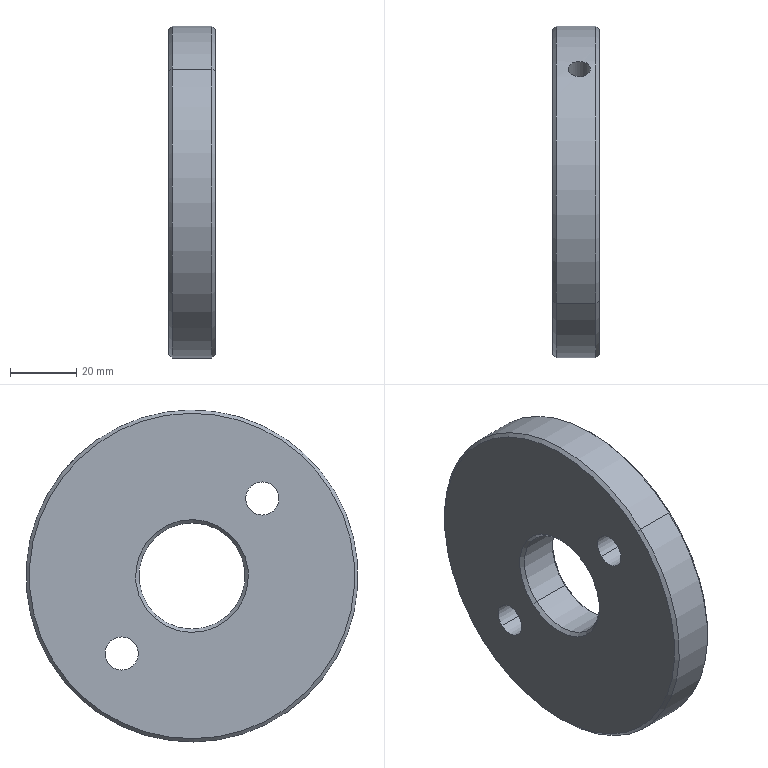Component | SolidWorks | 2-10-10WorkpieceAxisAssembly-1_Flange1-1 | 1 solid | 20 faces | box 14 x 100 x 100 mm | volume 94846 mm3 | cylinder 10 | cone 8 | plane 2 | commonest cylinder face diameters 10 x4 6.8 x2 32 x2 100 x2
STEP:
#1=COLOUR_RGB('',0.7922,0.8196,0.9333);
#2=FILL_AREA_STYLE_COLOUR('',#1);
#3=FILL_AREA_STYLE('',(#2));
#4=SURFACE_STYLE_FILL_AREA(#3);
#5=SURFACE_SIDE_STYLE('',(#4));
#6=SURFACE_STYLE_USAGE(.BOTH.,#5);
#7=PRESENTATION_STYLE_ASSIGNMENT((#6));
#8=CARTESIAN_POINT('',(-6.662,0.302,0.4232));
#9=VERTEX_POINT('',#8);
#10=CARTESIAN_POINT('',(-6.394,0.302,0.4232));
#11=VERTEX_POINT('',#10);
#12=CARTESIAN_POINT('',(-6.662,0.302,0.4232));
#13=CARTESIAN_POINT('',(-6.662,0.3079,0.4166));
#14=CARTESIAN_POINT('',(-6.661,0.3136,0.4101));
#15=CARTESIAN_POINT('',(-6.657,0.3246,0.3969));
#16=CARTESIAN_POINT('',(-6.655,0.33,0.3902));
#17=CARTESIAN_POINT('',(-6.648,0.3399,0.3773));
#18=CARTESIAN_POINT('',(-6.644,0.3444,0.3711));
#19=CARTESIAN_POINT('',(-6.634,0.3529,0.3592));
#20=CARTESIAN_POINT('',(-6.629,0.3568,0.3535));
#21=CARTESIAN_POINT('',(-6.616,0.3637,0.3431));
#22=CARTESIAN_POINT('',(-6.61,0.3667,0.3384));
#23=CARTESIAN_POINT('',(-6.595,0.372,0.3299));
#24=CARTESIAN_POINT('',(-6.587,0.3742,0.3263));
#25=CARTESIAN_POINT('',(-6.571,0.3777,0.3205));
#26=CARTESIAN_POINT('',(-6.563,0.379,0.3182));
#27=CARTESIAN_POINT('',(-6.545,0.3808,0.3152));
#28=CARTESIAN_POINT('',(-6.537,0.3812,0.3144));
#29=CARTESIAN_POINT('',(-6.519,0.3812,0.3144));
#30=CARTESIAN_POINT('',(-6.51,0.3808,0.3152));
#31=CARTESIAN_POINT('',(-6.493,0.379,0.3182));
#32=CARTESIAN_POINT('',(-6.485,0.3777,0.3205));
#33=CARTESIAN_POINT('',(-6.469,0.3742,0.3263));
#34=CARTESIAN_POINT('',(-6.461,0.372,0.33));
#35=CARTESIAN_POINT('',(-6.446,0.3668,0.3383));
#36=CARTESIAN_POINT('',(-6.439,0.3637,0.3431));
#37=CARTESIAN_POINT('',(-6.427,0.3568,0.3536));
#38=CARTESIAN_POINT('',(-6.422,0.3529,0.3592));
#39=CARTESIAN_POINT('',(-6.412,0.3445,0.371));
#40=CARTESIAN_POINT('',(-6.408,0.3398,0.3774));
#41=CARTESIAN_POINT('',(-6.401,0.3299,0.3903));
#42=CARTESIAN_POINT('',(-6.398,0.3247,0.3968));
#43=CARTESIAN_POINT('',(-6.395,0.3137,0.41));
#44=CARTESIAN_POINT('',(-6.394,0.3078,0.4167));
#45=CARTESIAN_POINT('',(-6.394,0.302,0.4232));
#46=B_SPLINE_CURVE_WITH_KNOTS('',3,(#12,#13,#14,#15,#16,#17,#18,#19,#20,#21,#22,#23,#24,#25,#26,#27,#28,#29,#30,#31,#32,#33,#34,#35,#36,#37,#38,#39,#40,#41,#42,#43,#44,#45),.UNSPECIFIED.,.F.,.F.,(4,2,2,2,2,2,2,2,2,2,2,2,2,2,2,2,4),(0.,0.0006663,0.001333,0.001999,0.002665,0.003331,0.003998,0.004664,0.00533,0.005996,0.006663,0.007329,0.007995,0.008662,0.009328,0.009994,0.01066),.UNSPECIFIED.);
#47=EDGE_CURVE('',#9,#11,#46,.T.);
#48=ORIENTED_EDGE('',*,*,#47,.T.);
#49=CARTESIAN_POINT('',(-6.394,1.293,1.323));
#50=VERTEX_POINT('',#49);
#51=CARTESIAN_POINT('',(-6.394,1.293,1.323));
#52=DIRECTION('',(0.,0.7407,0.6719));
#53=VECTOR('',#52,39.37);
#54=LINE('',#51,#53);
#55=EDGE_CURVE('',#11,#50,#54,.T.);
#56=ORIENTED_EDGE('',*,*,#55,.T.);
#57=CARTESIAN_POINT('',(-6.662,1.293,1.323));
#58=VERTEX_POINT('',#57);
#59=CARTESIAN_POINT('',(-6.662,1.293,1.323));
#60=CARTESIAN_POINT('',(-6.662,1.299,1.316));
#61=CARTESIAN_POINT('',(-6.661,1.305,1.31));
#62=CARTESIAN_POINT('',(-6.657,1.317,1.297));
#63=CARTESIAN_POINT('',(-6.655,1.322,1.29));
#64=CARTESIAN_POINT('',(-6.648,1.333,1.278));
#65=CARTESIAN_POINT('',(-6.644,1.338,1.272));
#66=CARTESIAN_POINT('',(-6.634,1.347,1.261));
#67=CARTESIAN_POINT('',(-6.629,1.351,1.256));
#68=CARTESIAN_POINT('',(-6.616,1.359,1.246));
#69=CARTESIAN_POINT('',(-6.61,1.363,1.242));
#70=CARTESIAN_POINT('',(-6.595,1.369,1.234));
#71=CARTESIAN_POINT('',(-6.587,1.372,1.231));
#72=CARTESIAN_POINT('',(-6.571,1.376,1.226));
#73=CARTESIAN_POINT('',(-6.563,1.377,1.224));
#74=CARTESIAN_POINT('',(-6.545,1.379,1.221));
#75=CARTESIAN_POINT('',(-6.537,1.38,1.22));
#76=CARTESIAN_POINT('',(-6.519,1.38,1.22));
#77=CARTESIAN_POINT('',(-6.51,1.379,1.221));
#78=CARTESIAN_POINT('',(-6.493,1.377,1.224));
#79=CARTESIAN_POINT('',(-6.485,1.376,1.226));
#80=CARTESIAN_POINT('',(-6.469,1.372,1.231));
#81=CARTESIAN_POINT('',(-6.461,1.369,1.234));
#82=CARTESIAN_POINT('',(-6.446,1.363,1.242));
#83=CARTESIAN_POINT('',(-6.44,1.359,1.246));
#84=CARTESIAN_POINT('',(-6.427,1.351,1.256));
#85=CARTESIAN_POINT('',(-6.421,1.347,1.261));
#86=CARTESIAN_POINT('',(-6.412,1.338,1.272));
#87=CARTESIAN_POINT('',(-6.408,1.333,1.278));
#88=CARTESIAN_POINT('',(-6.401,1.322,1.29));
#89=CARTESIAN_POINT('',(-6.398,1.317,1.297));
#90=CARTESIAN_POINT('',(-6.395,1.305,1.309));
#91=CARTESIAN_POINT('',(-6.394,1.299,1.316));
#92=CARTESIAN_POINT('',(-6.394,1.293,1.323));
#93=B_SPLINE_CURVE_WITH_KNOTS('',3,(#59,#60,#61,#62,#63,#64,#65,#66,#67,#68,#69,#70,#71,#72,#73,#74,#75,#76,#77,#78,#79,#80,#81,#82,#83,#84,#85,#86,#87,#88,#89,#90,#91,#92),.UNSPECIFIED.,.F.,.F.,(4,2,2,2,2,2,2,2,2,2,2,2,2,2,2,2,4),(0.,0.0006646,0.001329,0.001994,0.002658,0.003323,0.003987,0.004652,0.005317,0.005981,0.006646,0.00731,0.007975,0.008639,0.009304,0.009968,0.01063),.UNSPECIFIED.);
#94=EDGE_CURVE('',#58,#50,#93,.T.);
#95=ORIENTED_EDGE('',*,*,#94,.F.);
#96=CARTESIAN_POINT('',(-6.662,1.293,1.323));
#97=DIRECTION('',(0.,0.7407,0.6719));
#98=VECTOR('',#97,39.37);
#99=LINE('',#96,#98);
#100=EDGE_CURVE('',#9,#58,#99,.T.);
#101=ORIENTED_EDGE('',*,*,#100,.F.);
#102=EDGE_LOOP('',(#48,#56,#95,#101));
#103=FACE_OUTER_BOUND('',#102,.T.);
#104=CARTESIAN_POINT('',(-6.528,1.293,1.323));
#105=DIRECTION('',(0.,0.7407,0.6719));
#106=DIRECTION('',(-1.,0.,0.));
#107=AXIS2_PLACEMENT_3D('',#104,#105,#106);
#108=CYLINDRICAL_SURFACE('',#107,0.1339);
#109=ADVANCED_FACE('',(#103),#108,.F.);
#110=CARTESIAN_POINT('',(-6.843,-1.461,1.429));
#111=VERTEX_POINT('',#110);
#112=CARTESIAN_POINT('',(-6.843,1.131,-1.429));
#113=VERTEX_POINT('',#112);
#114=CARTESIAN_POINT('',(-6.843,-0.1646,-0.));
#115=DIRECTION('',(-1.,0.,-0.));
#116=DIRECTION('',(0.,-0.6719,0.7407));
#117=AXIS2_PLACEMENT_3D('',#114,#115,#116);
#118=CIRCLE('',#117,1.929);
#119=EDGE_CURVE('',#111,#113,#118,.T.);
#120=ORIENTED_EDGE('',*,*,#119,.F.);
#121=CARTESIAN_POINT('',(-6.804,-1.487,1.458));
#122=VERTEX_POINT('',#121);
#123=CARTESIAN_POINT('',(-6.843,-1.461,1.429));
#124=DIRECTION('',(0.7071,-0.4751,0.5237));
#125=VECTOR('',#124,39.37);
#126=LINE('',#123,#125);
#127=EDGE_CURVE('',#111,#122,#126,.T.);
#128=ORIENTED_EDGE('',*,*,#127,.T.);
#129=CARTESIAN_POINT('',(-6.804,1.158,-1.458));
#130=VERTEX_POINT('',#129);
#131=CARTESIAN_POINT('',(-6.804,-0.1646,-0.));
#132=DIRECTION('',(1.,-0.,0.));
#133=DIRECTION('',(0.,-0.6719,0.7407));
#134=AXIS2_PLACEMENT_3D('',#131,#132,#133);
#135=CIRCLE('',#134,1.969);
#136=EDGE_CURVE('',#130,#122,#135,.T.);
#137=ORIENTED_EDGE('',*,*,#136,.F.);
#138=CARTESIAN_POINT('',(-6.843,1.131,-1.429));
#139=DIRECTION('',(0.7071,0.4751,-0.5237));
#140=VECTOR('',#139,39.37);
#141=LINE('',#138,#140);
#142=EDGE_CURVE('',#113,#130,#141,.T.);
#143=ORIENTED_EDGE('',*,*,#142,.F.);
#144=EDGE_LOOP('',(#120,#128,#137,#143));
#145=FACE_OUTER_BOUND('',#144,.T.);
#146=CARTESIAN_POINT('',(-6.843,-0.1646,-0.));
#147=DIRECTION('',(1.,-0.,0.));
#148=DIRECTION('',(0.,0.6719,-0.7407));
#149=AXIS2_PLACEMENT_3D('',#146,#147,#148);
#150=CONICAL_SURFACE('',#149,1.929,0.7854);
#151=ADVANCED_FACE('',(#145),#150,.T.);
#152=CARTESIAN_POINT('',(-6.804,0.2586,-0.4666));
#153=VERTEX_POINT('',#152);
#154=CARTESIAN_POINT('',(-6.804,-0.5878,0.4666));
#155=VERTEX_POINT('',#154);
#156=CARTESIAN_POINT('',(-6.804,-0.1646,-0.));
#157=DIRECTION('',(-1.,0.,-0.));
#158=DIRECTION('',(0.,-0.6719,0.7407));
#159=AXIS2_PLACEMENT_3D('',#156,#157,#158);
#160=CIRCLE('',#159,0.6299);
#161=EDGE_CURVE('',#153,#155,#160,.T.);
#162=ORIENTED_EDGE('',*,*,#161,.F.);
#163=CARTESIAN_POINT('',(-6.843,0.2851,-0.4957));
#164=VERTEX_POINT('',#163);
#165=CARTESIAN_POINT('',(-6.804,0.2586,-0.4666));
#166=DIRECTION('',(-0.7071,0.4751,-0.5237));
#167=VECTOR('',#166,39.37);
#168=LINE('',#165,#167);
#169=EDGE_CURVE('',#153,#164,#168,.T.);
#170=ORIENTED_EDGE('',*,*,#169,.T.);
#171=CARTESIAN_POINT('',(-6.843,-0.6143,0.4957));
#172=VERTEX_POINT('',#171);
#173=CARTESIAN_POINT('',(-6.843,-0.1646,-0.));
#174=DIRECTION('',(1.,-0.,0.));
#175=DIRECTION('',(0.,-0.6719,0.7407));
#176=AXIS2_PLACEMENT_3D('',#173,#174,#175);
#177=CIRCLE('',#176,0.6693);
#178=EDGE_CURVE('',#172,#164,#177,.T.);
#179=ORIENTED_EDGE('',*,*,#178,.F.);
#180=CARTESIAN_POINT('',(-6.804,-0.5878,0.4666));
#181=DIRECTION('',(-0.7071,-0.4751,0.5237));
#182=VECTOR('',#181,39.37);
#183=LINE('',#180,#182);
#184=EDGE_CURVE('',#155,#172,#183,.T.);
#185=ORIENTED_EDGE('',*,*,#184,.F.);
#186=EDGE_LOOP('',(#162,#170,#179,#185));
#187=FACE_OUTER_BOUND('',#186,.T.);
#188=CARTESIAN_POINT('',(-6.804,-0.1646,-0.));
#189=DIRECTION('',(-1.,0.,-0.));
#190=DIRECTION('',(0.,-0.6719,0.7407));
#191=AXIS2_PLACEMENT_3D('',#188,#189,#190);
#192=CONICAL_SURFACE('',#191,0.6299,0.7854);
#193=ADVANCED_FACE('',(#187),#192,.F.);
#194=CARTESIAN_POINT('',(-6.292,1.131,-1.429));
#195=VERTEX_POINT('',#194);
#196=CARTESIAN_POINT('',(-6.292,-1.461,1.429));
#197=VERTEX_POINT('',#196);
#198=CARTESIAN_POINT('',(-6.292,-0.1646,-0.));
#199=DIRECTION('',(1.,-0.,0.));
#200=DIRECTION('',(0.,-0.6719,0.7407));
#201=AXIS2_PLACEMENT_3D('',#198,#199,#200);
#202=CIRCLE('',#201,1.929);
#203=EDGE_CURVE('',#195,#197,#202,.T.);
#204=ORIENTED_EDGE('',*,*,#203,.F.);
#205=CARTESIAN_POINT('',(-6.331,1.158,-1.458));
#206=VERTEX_POINT('',#205);
#207=CARTESIAN_POINT('',(-6.331,1.158,-1.458));
#208=DIRECTION('',(-0.7071,0.4751,-0.5237));
#209=VECTOR('',#208,39.37);
#210=LINE('',#207,#209);
#211=EDGE_CURVE('',#195,#206,#210,.T.);
#212=ORIENTED_EDGE('',*,*,#211,.T.);
#213=CARTESIAN_POINT('',(-6.331,-1.487,1.458));
#214=VERTEX_POINT('',#213);
#215=CARTESIAN_POINT('',(-6.331,-0.1646,-0.));
#216=DIRECTION('',(-1.,0.,-0.));
#217=DIRECTION('',(0.,-0.6719,0.7407));
#218=AXIS2_PLACEMENT_3D('',#215,#216,#217);
#219=CIRCLE('',#218,1.969);
#220=EDGE_CURVE('',#214,#206,#219,.T.);
#221=ORIENTED_EDGE('',*,*,#220,.F.);
#222=CARTESIAN_POINT('',(-6.331,-1.487,1.458));
#223=DIRECTION('',(-0.7071,-0.4751,0.5237));
#224=VECTOR('',#223,39.37);
#225=LINE('',#222,#224);
#226=EDGE_CURVE('',#197,#214,#225,.T.);
#227=ORIENTED_EDGE('',*,*,#226,.F.);
#228=EDGE_LOOP('',(#204,#212,#221,#227));
#229=FACE_OUTER_BOUND('',#228,.T.);
#230=CARTESIAN_POINT('',(-6.331,-0.1646,-0.));
#231=DIRECTION('',(-1.,0.,-0.));
#232=DIRECTION('',(0.,-0.6719,0.7407));
#233=AXIS2_PLACEMENT_3D('',#230,#231,#232);
#234=CONICAL_SURFACE('',#233,1.969,0.7854);
#235=ADVANCED_FACE('',(#229),#234,.T.);
#236=CARTESIAN_POINT('',(-6.331,-0.5878,0.4666));
#237=VERTEX_POINT('',#236);
#238=CARTESIAN_POINT('',(-6.331,0.2586,-0.4666));
#239=VERTEX_POINT('',#238);
#240=CARTESIAN_POINT('',(-6.331,-0.1646,-0.));
#241=DIRECTION('',(1.,-0.,0.));
#242=DIRECTION('',(0.,-0.6719,0.7407));
#243=AXIS2_PLACEMENT_3D('',#240,#241,#242);
#244=CIRCLE('',#243,0.6299);
#245=EDGE_CURVE('',#237,#239,#244,.T.);
#246=ORIENTED_EDGE('',*,*,#245,.F.);
#247=CARTESIAN_POINT('',(-6.292,-0.6143,0.4957));
#248=VERTEX_POINT('',#247);
#249=CARTESIAN_POINT('',(-6.292,-0.6143,0.4957));
#250=DIRECTION('',(0.7071,-0.4751,0.5237));
#251=VECTOR('',#250,39.37);
#252=LINE('',#249,#251);
#253=EDGE_CURVE('',#237,#248,#252,.T.);
#254=ORIENTED_EDGE('',*,*,#253,.T.);
#255=CARTESIAN_POINT('',(-6.292,0.2851,-0.4957));
#256=VERTEX_POINT('',#255);
#257=CARTESIAN_POINT('',(-6.292,-0.1646,-0.));
#258=DIRECTION('',(-1.,0.,-0.));
#259=DIRECTION('',(0.,-0.6719,0.7407));
#260=AXIS2_PLACEMENT_3D('',#257,#258,#259);
#261=CIRCLE('',#260,0.6693);
#262=EDGE_CURVE('',#256,#248,#261,.T.);
#263=ORIENTED_EDGE('',*,*,#262,.F.);
#264=CARTESIAN_POINT('',(-6.292,0.2851,-0.4957));
#265=DIRECTION('',(0.7071,0.4751,-0.5237));
#266=VECTOR('',#265,39.37);
#267=LINE('',#264,#266);
#268=EDGE_CURVE('',#239,#256,#267,.T.);
#269=ORIENTED_EDGE('',*,*,#268,.F.);
#270=EDGE_LOOP('',(#246,#254,#263,#269));
#271=FACE_OUTER_BOUND('',#270,.T.);
#272=CARTESIAN_POINT('',(-6.292,-0.1646,-0.));
#273=DIRECTION('',(1.,-0.,0.));
#274=DIRECTION('',(0.,0.6719,-0.7407));
#275=AXIS2_PLACEMENT_3D('',#272,#273,#274);
#276=CONICAL_SURFACE('',#275,0.6693,0.7854);
#277=ADVANCED_FACE('',(#271),#276,.F.);
#278=CARTESIAN_POINT('',(-6.843,-0.8656,0.7728));
#279=VERTEX_POINT('',#278);
#280=CARTESIAN_POINT('',(-6.843,-1.13,1.064));
#281=VERTEX_POINT('',#280);
#282=CARTESIAN_POINT('',(-6.843,-0.9978,0.9186));
#283=DIRECTION('',(-1.,0.,-0.));
#284=DIRECTION('',(0.,-0.6719,0.7407));
#285=AXIS2_PLACEMENT_3D('',#282,#283,#284);
#286=CIRCLE('',#285,0.1969);
#287=EDGE_CURVE('',#279,#281,#286,.T.);
#288=ORIENTED_EDGE('',*,*,#287,.T.);
#289=CARTESIAN_POINT('',(-6.292,-1.13,1.064));
#290=VERTEX_POINT('',#289);
#291=CARTESIAN_POINT('',(-6.843,-1.13,1.064));
#292=DIRECTION('',(1.,-0.,0.));
#293=VECTOR('',#292,39.37);
#294=LINE('',#291,#293);
#295=EDGE_CURVE('',#281,#290,#294,.T.);
#296=ORIENTED_EDGE('',*,*,#295,.T.);
#297=CARTESIAN_POINT('',(-6.292,-0.8656,0.7728));
#298=VERTEX_POINT('',#297);
#299=CARTESIAN_POINT('',(-6.292,-0.9978,0.9186));
#300=DIRECTION('',(-1.,0.,-0.));
#301=DIRECTION('',(0.,-0.6719,0.7407));
#302=AXIS2_PLACEMENT_3D('',#299,#300,#301);
#303=CIRCLE('',#302,0.1969);
#304=EDGE_CURVE('',#298,#290,#303,.T.);
#305=ORIENTED_EDGE('',*,*,#304,.F.);
#306=CARTESIAN_POINT('',(-6.843,-0.8656,0.7728));
#307=DIRECTION('',(1.,-0.,0.));
#308=VECTOR('',#307,39.37);
#309=LINE('',#306,#308);
#310=EDGE_CURVE('',#279,#298,#309,.T.);
#311=ORIENTED_EDGE('',*,*,#310,.F.);
#312=EDGE_LOOP('',(#288,#296,#305,#311));
#313=FACE_OUTER_BOUND('',#312,.T.);
#314=CARTESIAN_POINT('',(-6.843,-0.9978,0.9186));
#315=DIRECTION('',(1.,-0.,0.));
#316=DIRECTION('',(0.,0.6719,-0.7407));
#317=AXIS2_PLACEMENT_3D('',#314,#315,#316);
#318=CYLINDRICAL_SURFACE('',#317,0.1969);
#319=ADVANCED_FACE('',(#313),#318,.F.);
#320=CARTESIAN_POINT('',(-6.843,0.8009,-1.064));
#321=VERTEX_POINT('',#320);
#322=CARTESIAN_POINT('',(-6.843,0.5363,-0.7728));
#323=VERTEX_POINT('',#322);
#324=CARTESIAN_POINT('',(-6.843,0.6686,-0.9186));
#325=DIRECTION('',(-1.,0.,-0.));
#326=DIRECTION('',(0.,-0.6719,0.7407));
#327=AXIS2_PLACEMENT_3D('',#324,#325,#326);
#328=CIRCLE('',#327,0.1969);
#329=EDGE_CURVE('',#321,#323,#328,.T.);
#330=ORIENTED_EDGE('',*,*,#329,.T.);
#331=CARTESIAN_POINT('',(-6.292,0.5363,-0.7728));
#332=VERTEX_POINT('',#331);
#333=CARTESIAN_POINT('',(-6.843,0.5363,-0.7728));
#334=DIRECTION('',(1.,-0.,0.));
#335=VECTOR('',#334,39.37);
#336=LINE('',#333,#335);
#337=EDGE_CURVE('',#323,#332,#336,.T.);
#338=ORIENTED_EDGE('',*,*,#337,.T.);
#339=CARTESIAN_POINT('',(-6.292,0.8009,-1.064));
#340=VERTEX_POINT('',#339);
#341=CARTESIAN_POINT('',(-6.292,0.6686,-0.9186));
#342=DIRECTION('',(-1.,0.,-0.));
#343=DIRECTION('',(0.,-0.6719,0.7407));
#344=AXIS2_PLACEMENT_3D('',#341,#342,#343);
#345=CIRCLE('',#344,0.1969);
#346=EDGE_CURVE('',#340,#332,#345,.T.);
#347=ORIENTED_EDGE('',*,*,#346,.F.);
#348=CARTESIAN_POINT('',(-6.843,0.8009,-1.064));
#349=DIRECTION('',(1.,-0.,0.));
#350=VECTOR('',#349,39.37);
#351=LINE('',#348,#350);
#352=EDGE_CURVE('',#321,#340,#351,.T.);
#353=ORIENTED_EDGE('',*,*,#352,.F.);
#354=EDGE_LOOP('',(#330,#338,#347,#353));
#355=FACE_OUTER_BOUND('',#354,.T.);
#356=CARTESIAN_POINT('',(-6.843,0.6686,-0.9186));
#357=DIRECTION('',(1.,-0.,0.));
#358=DIRECTION('',(0.,0.6719,-0.7407));
#359=AXIS2_PLACEMENT_3D('',#356,#357,#358);
#360=CYLINDRICAL_SURFACE('',#359,0.1969);
#361=ADVANCED_FACE('',(#355),#360,.F.);
#362=ORIENTED_EDGE('',*,*,#161,.T.);
#363=CARTESIAN_POINT('',(-6.843,-0.5878,0.4666));
#364=DIRECTION('',(1.,-0.,0.));
#365=VECTOR('',#364,39.37);
#366=LINE('',#363,#365);
#367=EDGE_CURVE('',#155,#237,#366,.T.);
#368=ORIENTED_EDGE('',*,*,#367,.T.);
#369=ORIENTED_EDGE('',*,*,#245,.T.);
#370=CARTESIAN_POINT('',(-6.843,0.2586,-0.4666));
#371=DIRECTION('',(1.,-0.,0.));
#372=VECTOR('',#371,39.37);
#373=LINE('',#370,#372);
#374=EDGE_CURVE('',#153,#239,#373,.T.);
#375=ORIENTED_EDGE('',*,*,#374,.F.);
#376=EDGE_LOOP('',(#362,#368,#369,#375));
#377=FACE_OUTER_BOUND('',#376,.T.);
#378=CARTESIAN_POINT('',(-6.843,-0.1646,-0.));
#379=DIRECTION('',(1.,-0.,0.));
#380=DIRECTION('',(0.,0.6719,-0.7407));
#381=AXIS2_PLACEMENT_3D('',#378,#379,#380);
#382=CYLINDRICAL_SURFACE('',#381,0.6299);
#383=ADVANCED_FACE('',(#377),#382,.F.);
#384=ORIENTED_EDGE('',*,*,#94,.T.);
#385=CARTESIAN_POINT('',(-6.394,1.293,1.323));
#386=CARTESIAN_POINT('',(-6.394,1.288,1.329));
#387=CARTESIAN_POINT('',(-6.395,1.282,1.335));
#388=CARTESIAN_POINT('',(-6.398,1.27,1.348));
#389=CARTESIAN_POINT('',(-6.401,1.264,1.354));
#390=CARTESIAN_POINT('',(-6.408,1.253,1.366));
#391=CARTESIAN_POINT('',(-6.412,1.248,1.371));
#392=CARTESIAN_POINT('',(-6.421,1.237,1.382));
#393=CARTESIAN_POINT('',(-6.427,1.233,1.387));
#394=CARTESIAN_POINT('',(-6.439,1.224,1.395));
#395=CARTESIAN_POINT('',(-6.446,1.22,1.399));
#396=CARTESIAN_POINT('',(-6.461,1.213,1.406));
#397=CARTESIAN_POINT('',(-6.468,1.21,1.409));
#398=CARTESIAN_POINT('',(-6.485,1.205,1.414));
#399=CARTESIAN_POINT('',(-6.493,1.203,1.416));
#400=CARTESIAN_POINT('',(-6.51,1.201,1.418));
#401=CARTESIAN_POINT('',(-6.519,1.2,1.419));
#402=CARTESIAN_POINT('',(-6.537,1.2,1.419));
#403=CARTESIAN_POINT('',(-6.545,1.201,1.418));
#404=CARTESIAN_POINT('',(-6.562,1.203,1.416));
#405=CARTESIAN_POINT('',(-6.571,1.205,1.414));
#406=CARTESIAN_POINT('',(-6.587,1.21,1.409));
#407=CARTESIAN_POINT('',(-6.595,1.213,1.406));
#408=CARTESIAN_POINT('',(-6.609,1.22,1.4));
#409=CARTESIAN_POINT('',(-6.616,1.224,1.396));
#410=CARTESIAN_POINT('',(-6.629,1.232,1.387));
#411=CARTESIAN_POINT('',(-6.634,1.237,1.382));
#412=CARTESIAN_POINT('',(-6.644,1.247,1.372));
#413=CARTESIAN_POINT('',(-6.648,1.253,1.366));
#414=CARTESIAN_POINT('',(-6.658,1.27,1.349));
#415=CARTESIAN_POINT('',(-6.662,1.282,1.336));
#416=CARTESIAN_POINT('',(-6.662,1.293,1.323));
#417=B_SPLINE_CURVE_WITH_KNOTS('',3,(#385,#386,#387,#388,#389,#390,#391,#392,#393,#394,#395,#396,#397,#398,#399,#400,#401,#402,#403,#404,#405,#406,#407,#408,#409,#410,#411,#412,#413,#414,#415,#416),.UNSPECIFIED.,.F.,.F.,(4,2,2,2,2,2,2,2,2,2,2,2,2,2,2,4),(0.01063,0.0113,0.01196,0.01263,0.01329,0.01396,0.01462,0.01528,0.01595,0.01661,0.01728,0.01794,0.01861,0.01927,0.01993,0.02126),.UNSPECIFIED.);
#418=EDGE_CURVE('',#50,#58,#417,.T.);
#419=ORIENTED_EDGE('',*,*,#418,.T.);
#420=EDGE_LOOP('',(#384,#419));
#421=FACE_BOUND('',#420,.T.);
#422=ORIENTED_EDGE('',*,*,#136,.T.);
#423=CARTESIAN_POINT('',(-6.843,-1.487,1.458));
#424=DIRECTION('',(1.,-0.,0.));
#425=VECTOR('',#424,39.37);
#426=LINE('',#423,#425);
#427=EDGE_CURVE('',#122,#214,#426,.T.);
#428=ORIENTED_EDGE('',*,*,#427,.T.);
#429=ORIENTED_EDGE('',*,*,#220,.T.);
#430=CARTESIAN_POINT('',(-6.843,1.158,-1.458));
#431=DIRECTION('',(1.,-0.,0.));
#432=VECTOR('',#431,39.37);
#433=LINE('',#430,#432);
#434=EDGE_CURVE('',#130,#206,#433,.T.);
#435=ORIENTED_EDGE('',*,*,#434,.F.);
#436=EDGE_LOOP('',(#422,#428,#429,#435));
#437=FACE_OUTER_BOUND('',#436,.T.);
#438=CARTESIAN_POINT('',(-6.843,-0.1646,-0.));
#439=DIRECTION('',(1.,-0.,0.));
#440=DIRECTION('',(0.,0.6719,-0.7407));
#441=AXIS2_PLACEMENT_3D('',#438,#439,#440);
#442=CYLINDRICAL_SURFACE('',#441,1.969);
#443=ADVANCED_FACE('',(#421,#437),#442,.T.);
#444=ORIENTED_EDGE('',*,*,#178,.T.);
#445=CARTESIAN_POINT('',(-6.843,-0.1646,-0.));
#446=DIRECTION('',(1.,-0.,0.));
#447=DIRECTION('',(0.,-0.6719,0.7407));
#448=AXIS2_PLACEMENT_3D('',#445,#446,#447);
#449=CIRCLE('',#448,0.6693);
#450=EDGE_CURVE('',#164,#172,#449,.T.);
#451=ORIENTED_EDGE('',*,*,#450,.T.);
#452=EDGE_LOOP('',(#444,#451));
#453=FACE_BOUND('',#452,.T.);
#454=CARTESIAN_POINT('',(-6.843,-0.1646,-0.));
#455=DIRECTION('',(-1.,0.,-0.));
#456=DIRECTION('',(0.,-0.6719,0.7407));
#457=AXIS2_PLACEMENT_3D('',#454,#455,#456);
#458=CIRCLE('',#457,1.929);
#459=EDGE_CURVE('',#113,#111,#458,.T.);
#460=ORIENTED_EDGE('',*,*,#459,.T.);
#461=ORIENTED_EDGE('',*,*,#119,.T.);
#462=EDGE_LOOP('',(#460,#461));
#463=FACE_OUTER_BOUND('',#462,.T.);
#464=ORIENTED_EDGE('',*,*,#329,.F.);
#465=CARTESIAN_POINT('',(-6.843,0.6686,-0.9186));
#466=DIRECTION('',(-1.,0.,-0.));
#467=DIRECTION('',(0.,-0.6719,0.7407));
#468=AXIS2_PLACEMENT_3D('',#465,#466,#467);
#469=CIRCLE('',#468,0.1969);
#470=EDGE_CURVE('',#323,#321,#469,.T.);
#471=ORIENTED_EDGE('',*,*,#470,.F.);
#472=EDGE_LOOP('',(#464,#471));
#473=FACE_BOUND('',#472,.T.);
#474=ORIENTED_EDGE('',*,*,#287,.F.);
#475=CARTESIAN_POINT('',(-6.843,-0.9978,0.9186));
#476=DIRECTION('',(-1.,0.,-0.));
#477=DIRECTION('',(0.,-0.6719,0.7407));
#478=AXIS2_PLACEMENT_3D('',#475,#476,#477);
#479=CIRCLE('',#478,0.1969);
#480=EDGE_CURVE('',#281,#279,#479,.T.);
#481=ORIENTED_EDGE('',*,*,#480,.F.);
#482=EDGE_LOOP('',(#474,#481));
#483=FACE_BOUND('',#482,.T.);
#484=CARTESIAN_POINT('',(-6.843,-0.1646,-0.));
#485=DIRECTION('',(-1.,0.,-0.));
#486=DIRECTION('',(-0.,-0.6719,0.7407));
#487=AXIS2_PLACEMENT_3D('',#484,#485,#486);
#488=PLANE('',#487);
#489=ADVANCED_FACE('',(#453,#463,#473,#483),#488,.T.);
#490=ORIENTED_EDGE('',*,*,#262,.T.);
#491=CARTESIAN_POINT('',(-6.292,-0.1646,-0.));
#492=DIRECTION('',(-1.,0.,-0.));
#493=DIRECTION('',(0.,-0.6719,0.7407));
#494=AXIS2_PLACEMENT_3D('',#491,#492,#493);
#495=CIRCLE('',#494,0.6693);
#496=EDGE_CURVE('',#248,#256,#495,.T.);
#497=ORIENTED_EDGE('',*,*,#496,.T.);
#498=EDGE_LOOP('',(#490,#497));
#499=FACE_BOUND('',#498,.T.);
#500=CARTESIAN_POINT('',(-6.292,-0.1646,-0.));
#501=DIRECTION('',(1.,-0.,0.));
#502=DIRECTION('',(0.,-0.6719,0.7407));
#503=AXIS2_PLACEMENT_3D('',#500,#501,#502);
#504=CIRCLE('',#503,1.929);
#505=EDGE_CURVE('',#197,#195,#504,.T.);
#506=ORIENTED_EDGE('',*,*,#505,.T.);
#507=ORIENTED_EDGE('',*,*,#203,.T.);
#508=EDGE_LOOP('',(#506,#507));
#509=FACE_OUTER_BOUND('',#508,.T.);
#510=ORIENTED_EDGE('',*,*,#346,.T.);
#511=CARTESIAN_POINT('',(-6.292,0.6686,-0.9186));
#512=DIRECTION('',(-1.,0.,-0.));
#513=DIRECTION('',(0.,-0.6719,0.7407));
#514=AXIS2_PLACEMENT_3D('',#511,#512,#513);
#515=CIRCLE('',#514,0.1969);
#516=EDGE_CURVE('',#332,#340,#515,.T.);
#517=ORIENTED_EDGE('',*,*,#516,.T.);
#518=EDGE_LOOP('',(#510,#517));
#519=FACE_BOUND('',#518,.T.);
#520=ORIENTED_EDGE('',*,*,#304,.T.);
#521=CARTESIAN_POINT('',(-6.292,-0.9978,0.9186));
#522=DIRECTION('',(-1.,0.,-0.));
#523=DIRECTION('',(0.,-0.6719,0.7407));
#524=AXIS2_PLACEMENT_3D('',#521,#522,#523);
#525=CIRCLE('',#524,0.1969);
#526=EDGE_CURVE('',#290,#298,#525,.T.);
#527=ORIENTED_EDGE('',*,*,#526,.T.);
#528=EDGE_LOOP('',(#520,#527));
#529=FACE_BOUND('',#528,.T.);
#530=CARTESIAN_POINT('',(-6.292,-0.1646,-0.));
#531=DIRECTION('',(-1.,0.,-0.));
#532=DIRECTION('',(-0.,-0.6719,0.7407));
#533=AXIS2_PLACEMENT_3D('',#530,#531,#532);
#534=PLANE('',#533);
#535=ADVANCED_FACE('',(#499,#509,#519,#529),#534,.F.);
#536=ORIENTED_EDGE('',*,*,#427,.F.);
#537=CARTESIAN_POINT('',(-6.804,-0.1646,-0.));
#538=DIRECTION('',(1.,-0.,0.));
#539=DIRECTION('',(0.,-0.6719,0.7407));
#540=AXIS2_PLACEMENT_3D('',#537,#538,#539);
#541=CIRCLE('',#540,1.969);
#542=EDGE_CURVE('',#122,#130,#541,.T.);
#543=ORIENTED_EDGE('',*,*,#542,.T.);
#544=ORIENTED_EDGE('',*,*,#434,.T.);
#545=CARTESIAN_POINT('',(-6.331,-0.1646,-0.));
#546=DIRECTION('',(-1.,0.,-0.));
#547=DIRECTION('',(0.,-0.6719,0.7407));
#548=AXIS2_PLACEMENT_3D('',#545,#546,#547);
#549=CIRCLE('',#548,1.969);
#550=EDGE_CURVE('',#206,#214,#549,.T.);
#551=ORIENTED_EDGE('',*,*,#550,.T.);
#552=EDGE_LOOP('',(#536,#543,#544,#551));
#553=FACE_OUTER_BOUND('',#552,.T.);
#554=CARTESIAN_POINT('',(-6.843,-0.1646,-0.));
#555=DIRECTION('',(1.,-0.,0.));
#556=DIRECTION('',(0.,0.6719,-0.7407));
#557=AXIS2_PLACEMENT_3D('',#554,#555,#556);
#558=CYLINDRICAL_SURFACE('',#557,1.969);
#559=ADVANCED_FACE('',(#553),#558,.T.);
#560=ORIENTED_EDGE('',*,*,#367,.F.);
#561=CARTESIAN_POINT('',(-6.804,-0.1646,-0.));
#562=DIRECTION('',(-1.,0.,-0.));
#563=DIRECTION('',(0.,-0.6719,0.7407));
#564=AXIS2_PLACEMENT_3D('',#561,#562,#563);
#565=CIRCLE('',#564,0.6299);
#566=EDGE_CURVE('',#155,#153,#565,.T.);
#567=ORIENTED_EDGE('',*,*,#566,.T.);
#568=ORIENTED_EDGE('',*,*,#374,.T.);
#569=CARTESIAN_POINT('',(-6.331,-0.1646,-0.));
#570=DIRECTION('',(1.,-0.,0.));
#571=DIRECTION('',(0.,-0.6719,0.7407));
#572=AXIS2_PLACEMENT_3D('',#569,#570,#571);
#573=CIRCLE('',#572,0.6299);
#574=EDGE_CURVE('',#239,#237,#573,.T.);
#575=ORIENTED_EDGE('',*,*,#574,.T.);
#576=EDGE_LOOP('',(#560,#567,#568,#575));
#577=FACE_OUTER_BOUND('',#576,.T.);
#578=ORIENTED_EDGE('',*,*,#47,.F.);
#579=CARTESIAN_POINT('',(-6.394,0.302,0.4232));
#580=CARTESIAN_POINT('',(-6.394,0.2961,0.4297));
#581=CARTESIAN_POINT('',(-6.395,0.2901,0.436));
#582=CARTESIAN_POINT('',(-6.398,0.2779,0.4484));
#583=CARTESIAN_POINT('',(-6.401,0.2719,0.4543));
#584=CARTESIAN_POINT('',(-6.408,0.2601,0.4653));
#585=CARTESIAN_POINT('',(-6.412,0.2542,0.4706));
#586=CARTESIAN_POINT('',(-6.422,0.2432,0.4802));
#587=CARTESIAN_POINT('',(-6.427,0.238,0.4845));
#588=CARTESIAN_POINT('',(-6.439,0.2283,0.4924));
#589=CARTESIAN_POINT('',(-6.446,0.2238,0.496));
#590=CARTESIAN_POINT('',(-6.461,0.216,0.502));
#591=CARTESIAN_POINT('',(-6.468,0.2126,0.5045));
#592=CARTESIAN_POINT('',(-6.493,0.2043,0.5106));
#593=CARTESIAN_POINT('',(-6.51,0.2014,0.5127));
#594=CARTESIAN_POINT('',(-6.537,0.2014,0.5127));
#595=CARTESIAN_POINT('',(-6.545,0.2021,0.5122));
#596=CARTESIAN_POINT('',(-6.563,0.2049,0.5102));
#597=CARTESIAN_POINT('',(-6.571,0.2071,0.5086));
#598=CARTESIAN_POINT('',(-6.587,0.2126,0.5045));
#599=CARTESIAN_POINT('',(-6.595,0.2159,0.502));
#600=CARTESIAN_POINT('',(-6.61,0.2237,0.496));
#601=CARTESIAN_POINT('',(-6.616,0.2282,0.4925));
#602=CARTESIAN_POINT('',(-6.629,0.2378,0.4846));
#603=CARTESIAN_POINT('',(-6.634,0.2431,0.4803));
#604=CARTESIAN_POINT('',(-6.644,0.2542,0.4706));
#605=CARTESIAN_POINT('',(-6.648,0.2599,0.4654));
#606=CARTESIAN_POINT('',(-6.655,0.2717,0.4544));
#607=CARTESIAN_POINT('',(-6.657,0.2779,0.4484));
#608=CARTESIAN_POINT('',(-6.661,0.29,0.4361));
#609=CARTESIAN_POINT('',(-6.662,0.296,0.4298));
#610=CARTESIAN_POINT('',(-6.662,0.302,0.4232));
#611=B_SPLINE_CURVE_WITH_KNOTS('',3,(#579,#580,#581,#582,#583,#584,#585,#586,#587,#588,#589,#590,#591,#592,#593,#594,#595,#596,#597,#598,#599,#600,#601,#602,#603,#604,#605,#606,#607,#608,#609,#610),.UNSPECIFIED.,.F.,.F.,(4,2,2,2,2,2,2,2,2,2,2,2,2,2,2,4),(0.01066,0.01133,0.01199,0.01266,0.01332,0.01399,0.01466,0.01599,0.01666,0.01732,0.01799,0.01865,0.01932,0.01999,0.02065,0.02132),.UNSPECIFIED.);
#612=EDGE_CURVE('',#11,#9,#611,.T.);
#613=ORIENTED_EDGE('',*,*,#612,.F.);
#614=EDGE_LOOP('',(#578,#613));
#615=FACE_BOUND('',#614,.T.);
#616=CARTESIAN_POINT('',(-6.843,-0.1646,-0.));
#617=DIRECTION('',(1.,-0.,0.));
#618=DIRECTION('',(0.,0.6719,-0.7407));
#619=AXIS2_PLACEMENT_3D('',#616,#617,#618);
#620=CYLINDRICAL_SURFACE('',#619,0.6299);
#621=ADVANCED_FACE('',(#577,#615),#620,.F.);
#622=ORIENTED_EDGE('',*,*,#337,.F.);
#623=ORIENTED_EDGE('',*,*,#470,.T.);
#624=ORIENTED_EDGE('',*,*,#352,.T.);
#625=ORIENTED_EDGE('',*,*,#516,.F.);
#626=EDGE_LOOP('',(#622,#623,#624,#625));
#627=FACE_OUTER_BOUND('',#626,.T.);
#628=CARTESIAN_POINT('',(-6.843,0.6686,-0.9186));
#629=DIRECTION('',(1.,-0.,0.));
#630=DIRECTION('',(0.,0.6719,-0.7407));
#631=AXIS2_PLACEMENT_3D('',#628,#629,#630);
#632=CYLINDRICAL_SURFACE('',#631,0.1969);
#633=ADVANCED_FACE('',(#627),#632,.F.);
#634=ORIENTED_EDGE('',*,*,#295,.F.);
#635=ORIENTED_EDGE('',*,*,#480,.T.);
#636=ORIENTED_EDGE('',*,*,#310,.T.);
#637=ORIENTED_EDGE('',*,*,#526,.F.);
#638=EDGE_LOOP('',(#634,#635,#636,#637));
#639=FACE_OUTER_BOUND('',#638,.T.);
#640=CARTESIAN_POINT('',(-6.843,-0.9978,0.9186));
#641=DIRECTION('',(1.,-0.,0.));
#642=DIRECTION('',(0.,0.6719,-0.7407));
#643=AXIS2_PLACEMENT_3D('',#640,#641,#642);
#644=CYLINDRICAL_SURFACE('',#643,0.1969);
#645=ADVANCED_FACE('',(#639),#644,.F.);
#646=ORIENTED_EDGE('',*,*,#253,.F.);
#647=ORIENTED_EDGE('',*,*,#574,.F.);
#648=ORIENTED_EDGE('',*,*,#268,.T.);
#649=ORIENTED_EDGE('',*,*,#496,.F.);
#650=EDGE_LOOP('',(#646,#647,#648,#649));
#651=FACE_OUTER_BOUND('',#650,.T.);
#652=CARTESIAN_POINT('',(-6.292,-0.1646,-0.));
#653=DIRECTION('',(1.,-0.,0.));
#654=DIRECTION('',(0.,0.6719,-0.7407));
#655=AXIS2_PLACEMENT_3D('',#652,#653,#654);
#656=CONICAL_SURFACE('',#655,0.6693,0.7854);
#657=ADVANCED_FACE('',(#651),#656,.F.);
#658=ORIENTED_EDGE('',*,*,#211,.F.);
#659=ORIENTED_EDGE('',*,*,#505,.F.);
#660=ORIENTED_EDGE('',*,*,#226,.T.);
#661=ORIENTED_EDGE('',*,*,#550,.F.);
#662=EDGE_LOOP('',(#658,#659,#660,#661));
#663=FACE_OUTER_BOUND('',#662,.T.);
#664=CARTESIAN_POINT('',(-6.331,-0.1646,-0.));
#665=DIRECTION('',(-1.,0.,-0.));
#666=DIRECTION('',(0.,-0.6719,0.7407));
#667=AXIS2_PLACEMENT_3D('',#664,#665,#666);
#668=CONICAL_SURFACE('',#667,1.969,0.7854);
#669=ADVANCED_FACE('',(#663),#668,.T.);
#670=ORIENTED_EDGE('',*,*,#169,.F.);
#671=ORIENTED_EDGE('',*,*,#566,.F.);
#672=ORIENTED_EDGE('',*,*,#184,.T.);
#673=ORIENTED_EDGE('',*,*,#450,.F.);
#674=EDGE_LOOP('',(#670,#671,#672,#673));
#675=FACE_OUTER_BOUND('',#674,.T.);
#676=CARTESIAN_POINT('',(-6.804,-0.1646,-0.));
#677=DIRECTION('',(-1.,0.,-0.));
#678=DIRECTION('',(0.,-0.6719,0.7407));
#679=AXIS2_PLACEMENT_3D('',#676,#677,#678);
#680=CONICAL_SURFACE('',#679,0.6299,0.7854);
#681=ADVANCED_FACE('',(#675),#680,.F.);
#682=ORIENTED_EDGE('',*,*,#127,.F.);
#683=ORIENTED_EDGE('',*,*,#459,.F.);
#684=ORIENTED_EDGE('',*,*,#142,.T.);
#685=ORIENTED_EDGE('',*,*,#542,.F.);
#686=EDGE_LOOP('',(#682,#683,#684,#685));
#687=FACE_OUTER_BOUND('',#686,.T.);
#688=CARTESIAN_POINT('',(-6.843,-0.1646,-0.));
#689=DIRECTION('',(1.,-0.,0.));
#690=DIRECTION('',(0.,0.6719,-0.7407));
#691=AXIS2_PLACEMENT_3D('',#688,#689,#690);
#692=CONICAL_SURFACE('',#691,1.929,0.7854);
#693=ADVANCED_FACE('',(#687),#692,.T.);
#694=ORIENTED_EDGE('',*,*,#55,.F.);
#695=ORIENTED_EDGE('',*,*,#612,.T.);
#696=ORIENTED_EDGE('',*,*,#100,.T.);
#697=ORIENTED_EDGE('',*,*,#418,.F.);
#698=EDGE_LOOP('',(#694,#695,#696,#697));
#699=FACE_OUTER_BOUND('',#698,.T.);
#700=CARTESIAN_POINT('',(-6.528,1.293,1.323));
#701=DIRECTION('',(0.,0.7407,0.6719));
#702=DIRECTION('',(-1.,0.,0.));
#703=AXIS2_PLACEMENT_3D('',#700,#701,#702);
#704=CYLINDRICAL_SURFACE('',#703,0.1339);
#705=ADVANCED_FACE('',(#699),#704,.F.);
#706=CLOSED_SHELL('',(#109,#151,#193,#235,#277,#319,#361,#383,#443,#489,#535,#559,#621,#633,#645,#657,#669,#681,#693,#705));
#707=MANIFOLD_SOLID_BREP('',#706);
#708=STYLED_ITEM('',(#7),#707);
#709=PRESENTATION_LAYER_ASSIGNMENT('','',(#708));
#710=CARTESIAN_POINT('',(0.,0.,0.));
#711=DIRECTION('',(0.,0.,1.));
#712=DIRECTION('',(1.,0.,0.));
#713=AXIS2_PLACEMENT_3D('',#710,#711,#712);
#714=(LENGTH_UNIT()NAMED_UNIT(*)SI_UNIT($,.METRE.));
#715=LENGTH_MEASURE_WITH_UNIT(LENGTH_MEASURE(0.0254),#714);
#716=DIMENSIONAL_EXPONENTS(1.,0.,0.,0.,0.,0.,0.);
#717=(CONVERSION_BASED_UNIT('',#715)LENGTH_UNIT()NAMED_UNIT(#716));
#718=UNCERTAINTY_MEASURE_WITH_UNIT(LENGTH_MEASURE(0.00001),#717,'','');
#719=(NAMED_UNIT(*)PLANE_ANGLE_UNIT()SI_UNIT($,.RADIAN.));
#720=(NAMED_UNIT(*)SI_UNIT($,.STERADIAN.)SOLID_ANGLE_UNIT());
#721=(GEOMETRIC_REPRESENTATION_CONTEXT(3)GLOBAL_UNCERTAINTY_ASSIGNED_CONTEXT((#718))GLOBAL_UNIT_ASSIGNED_CONTEXT((#717,#719,#720))REPRESENTATION_CONTEXT('',''));
#722=ADVANCED_BREP_SHAPE_REPRESENTATION('',(#707,#713),#721);
#723=(LENGTH_UNIT()NAMED_UNIT(*)SI_UNIT($,.METRE.));
#724=LENGTH_MEASURE_WITH_UNIT(LENGTH_MEASURE(0.0254),#723);
#725=DIMENSIONAL_EXPONENTS(1.,0.,0.,0.,0.,0.,0.);
#726=(CONVERSION_BASED_UNIT('',#724)LENGTH_UNIT()NAMED_UNIT(#725));
#727=UNCERTAINTY_MEASURE_WITH_UNIT(LENGTH_MEASURE(0.00001),#726,'','');
#728=(NAMED_UNIT(*)PLANE_ANGLE_UNIT()SI_UNIT($,.RADIAN.));
#729=(NAMED_UNIT(*)SI_UNIT($,.STERADIAN.)SOLID_ANGLE_UNIT());
#730=(GEOMETRIC_REPRESENTATION_CONTEXT(3)GLOBAL_UNCERTAINTY_ASSIGNED_CONTEXT((#727))GLOBAL_UNIT_ASSIGNED_CONTEXT((#726,#728,#729))REPRESENTATION_CONTEXT('',''));
#731=MECHANICAL_DESIGN_GEOMETRIC_PRESENTATION_REPRESENTATION('',(#708),#730);